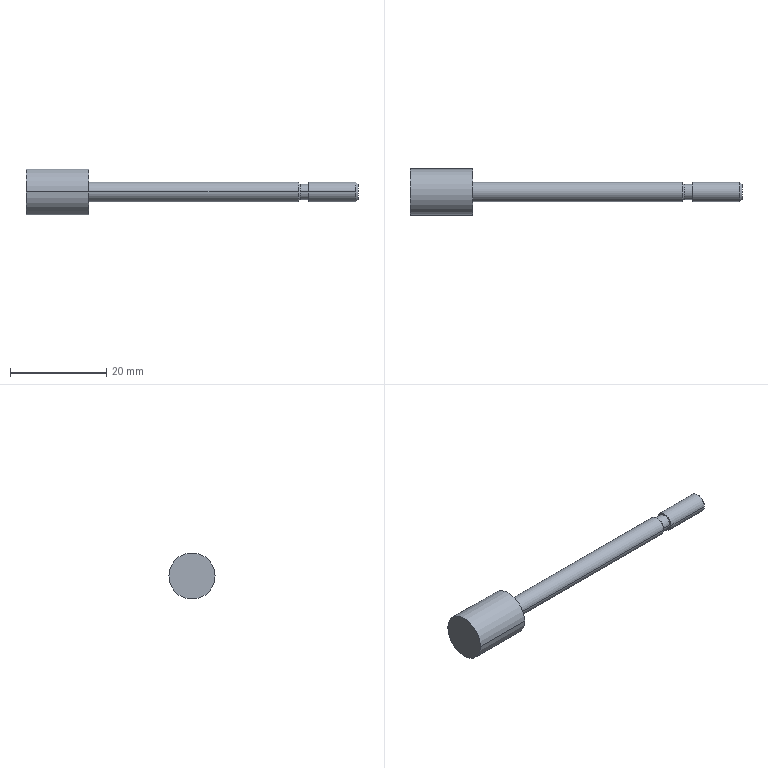Component | SolidWorks | MI10x10U(0)+()-1_MI 10x10-U_r-1 | 1 solid | 16 faces | box 69 x 9.6 x 9.6 mm | volume 1635 mm3 | cylinder 8 | cone 4 | plane 4 | commonest cylinder face diameters 4 x4 9.6 x2 3.2 x2
build123d program:
from build123d import *


with BuildPart() as part:
    # Sketch1 → Revolve1 (revolve)
    with BuildSketch(Plane.XY, mode=Mode.PRIVATE) as revolve1_sk:
        Polygon((-28, 0), (-28, 1.571), (-27.57, 2), (-17.8, 2), (-17.8, 1.6), (-16, 1.6), (-15.6, 2), (28, 2), (28, 4.8), (41, 4.8), (41, 0), align=None)
    revolve(revolve1_sk.sketch.rotate(Axis((41, 0, 0), (-1, 0, 0)), 270), axis=Axis((41, 0, 0), (-1, 0, 0)))


solid = part.part

# Placed as in the assembly
solid = solid.moved(Location((-19.294, 30.452, 72.77), (-180, 0, 180)))
STEP:
#1=COLOUR_RGB('',0.7922,0.8196,0.9333);
#2=FILL_AREA_STYLE_COLOUR('',#1);
#3=FILL_AREA_STYLE('',(#2));
#4=SURFACE_STYLE_FILL_AREA(#3);
#5=SURFACE_SIDE_STYLE('',(#4));
#6=SURFACE_STYLE_USAGE(.BOTH.,#5);
#7=PRESENTATION_STYLE_ASSIGNMENT((#6));
#8=CARTESIAN_POINT('',(-2.374,1.388,2.865));
#9=VERTEX_POINT('',#8);
#10=CARTESIAN_POINT('',(-2.374,1.01,2.865));
#11=VERTEX_POINT('',#10);
#12=CARTESIAN_POINT('',(-2.374,1.199,2.865));
#13=DIRECTION('',(1.,-0.,-0.));
#14=DIRECTION('',(0.,1.,0.));
#15=AXIS2_PLACEMENT_3D('',#12,#13,#14);
#16=CIRCLE('',#15,0.189);
#17=EDGE_CURVE('',#9,#11,#16,.T.);
#18=ORIENTED_EDGE('',*,*,#17,.T.);
#19=CARTESIAN_POINT('',(-1.862,1.01,2.865));
#20=VERTEX_POINT('',#19);
#21=CARTESIAN_POINT('',(-2.374,1.01,2.865));
#22=DIRECTION('',(1.,-0.,-0.));
#23=VECTOR('',#22,39.37);
#24=LINE('',#21,#23);
#25=EDGE_CURVE('',#11,#20,#24,.T.);
#26=ORIENTED_EDGE('',*,*,#25,.T.);
#27=CARTESIAN_POINT('',(-1.862,1.388,2.865));
#28=VERTEX_POINT('',#27);
#29=CARTESIAN_POINT('',(-1.862,1.199,2.865));
#30=DIRECTION('',(1.,-0.,-0.));
#31=DIRECTION('',(0.,1.,0.));
#32=AXIS2_PLACEMENT_3D('',#29,#30,#31);
#33=CIRCLE('',#32,0.189);
#34=EDGE_CURVE('',#28,#20,#33,.T.);
#35=ORIENTED_EDGE('',*,*,#34,.F.);
#36=CARTESIAN_POINT('',(-2.374,1.388,2.865));
#37=DIRECTION('',(1.,-0.,-0.));
#38=VECTOR('',#37,39.37);
#39=LINE('',#36,#38);
#40=EDGE_CURVE('',#9,#28,#39,.T.);
#41=ORIENTED_EDGE('',*,*,#40,.F.);
#42=EDGE_LOOP('',(#18,#26,#35,#41));
#43=FACE_OUTER_BOUND('',#42,.T.);
#44=CARTESIAN_POINT('',(-2.374,1.199,2.865));
#45=DIRECTION('',(1.,-0.,-0.));
#46=DIRECTION('',(0.,1.,0.));
#47=AXIS2_PLACEMENT_3D('',#44,#45,#46);
#48=CYLINDRICAL_SURFACE('',#47,0.189);
#49=ADVANCED_FACE('',(#43),#48,.T.);
#50=CARTESIAN_POINT('',(-1.862,1.278,2.865));
#51=VERTEX_POINT('',#50);
#52=CARTESIAN_POINT('',(-1.862,1.12,2.865));
#53=VERTEX_POINT('',#52);
#54=CARTESIAN_POINT('',(-1.862,1.199,2.865));
#55=DIRECTION('',(1.,-0.,-0.));
#56=DIRECTION('',(0.,1.,0.));
#57=AXIS2_PLACEMENT_3D('',#54,#55,#56);
#58=CIRCLE('',#57,0.07874);
#59=EDGE_CURVE('',#51,#53,#58,.T.);
#60=ORIENTED_EDGE('',*,*,#59,.T.);
#61=CARTESIAN_POINT('',(-0.1454,1.12,2.865));
#62=VERTEX_POINT('',#61);
#63=CARTESIAN_POINT('',(-2.374,1.12,2.865));
#64=DIRECTION('',(1.,-0.,-0.));
#65=VECTOR('',#64,39.37);
#66=LINE('',#63,#65);
#67=EDGE_CURVE('',#53,#62,#66,.T.);
#68=ORIENTED_EDGE('',*,*,#67,.T.);
#69=CARTESIAN_POINT('',(-0.1454,1.278,2.865));
#70=VERTEX_POINT('',#69);
#71=CARTESIAN_POINT('',(-0.1454,1.199,2.865));
#72=DIRECTION('',(1.,-0.,-0.));
#73=DIRECTION('',(0.,1.,0.));
#74=AXIS2_PLACEMENT_3D('',#71,#72,#73);
#75=CIRCLE('',#74,0.07874);
#76=EDGE_CURVE('',#70,#62,#75,.T.);
#77=ORIENTED_EDGE('',*,*,#76,.F.);
#78=CARTESIAN_POINT('',(-2.374,1.278,2.865));
#79=DIRECTION('',(1.,-0.,-0.));
#80=VECTOR('',#79,39.37);
#81=LINE('',#78,#80);
#82=EDGE_CURVE('',#51,#70,#81,.T.);
#83=ORIENTED_EDGE('',*,*,#82,.F.);
#84=EDGE_LOOP('',(#60,#68,#77,#83));
#85=FACE_OUTER_BOUND('',#84,.T.);
#86=CARTESIAN_POINT('',(-2.374,1.199,2.865));
#87=DIRECTION('',(1.,-0.,-0.));
#88=DIRECTION('',(0.,1.,0.));
#89=AXIS2_PLACEMENT_3D('',#86,#87,#88);
#90=CYLINDRICAL_SURFACE('',#89,0.07874);
#91=ADVANCED_FACE('',(#85),#90,.T.);
#92=CARTESIAN_POINT('',(-0.1297,1.262,2.865));
#93=VERTEX_POINT('',#92);
#94=CARTESIAN_POINT('',(-0.1297,1.136,2.865));
#95=VERTEX_POINT('',#94);
#96=CARTESIAN_POINT('',(-0.1297,1.199,2.865));
#97=DIRECTION('',(1.,-0.,-0.));
#98=DIRECTION('',(0.,1.,0.));
#99=AXIS2_PLACEMENT_3D('',#96,#97,#98);
#100=CIRCLE('',#99,0.06299);
#101=EDGE_CURVE('',#93,#95,#100,.T.);
#102=ORIENTED_EDGE('',*,*,#101,.F.);
#103=CARTESIAN_POINT('',(-0.1454,1.278,2.865));
#104=DIRECTION('',(-0.7071,0.7071,0.));
#105=VECTOR('',#104,39.37);
#106=LINE('',#103,#105);
#107=EDGE_CURVE('',#93,#70,#106,.T.);
#108=ORIENTED_EDGE('',*,*,#107,.T.);
#109=ORIENTED_EDGE('',*,*,#76,.T.);
#110=CARTESIAN_POINT('',(-0.1454,1.12,2.865));
#111=DIRECTION('',(-0.7071,-0.7071,-0.));
#112=VECTOR('',#111,39.37);
#113=LINE('',#110,#112);
#114=EDGE_CURVE('',#95,#62,#113,.T.);
#115=ORIENTED_EDGE('',*,*,#114,.F.);
#116=EDGE_LOOP('',(#102,#108,#109,#115));
#117=FACE_OUTER_BOUND('',#116,.T.);
#118=CARTESIAN_POINT('',(-0.1454,1.199,2.865));
#119=DIRECTION('',(-1.,0.,0.));
#120=DIRECTION('',(-0.,-1.,0.));
#121=AXIS2_PLACEMENT_3D('',#118,#119,#120);
#122=CONICAL_SURFACE('',#121,0.07874,0.7854);
#123=ADVANCED_FACE('',(#117),#122,.T.);
#124=ORIENTED_EDGE('',*,*,#101,.T.);
#125=CARTESIAN_POINT('',(-0.05882,1.136,2.865));
#126=VERTEX_POINT('',#125);
#127=CARTESIAN_POINT('',(-2.374,1.136,2.865));
#128=DIRECTION('',(1.,-0.,-0.));
#129=VECTOR('',#128,39.37);
#130=LINE('',#127,#129);
#131=EDGE_CURVE('',#95,#126,#130,.T.);
#132=ORIENTED_EDGE('',*,*,#131,.T.);
#133=CARTESIAN_POINT('',(-0.05882,1.262,2.865));
#134=VERTEX_POINT('',#133);
#135=CARTESIAN_POINT('',(-0.05882,1.199,2.865));
#136=DIRECTION('',(1.,-0.,-0.));
#137=DIRECTION('',(0.,1.,0.));
#138=AXIS2_PLACEMENT_3D('',#135,#136,#137);
#139=CIRCLE('',#138,0.06299);
#140=EDGE_CURVE('',#134,#126,#139,.T.);
#141=ORIENTED_EDGE('',*,*,#140,.F.);
#142=CARTESIAN_POINT('',(-2.374,1.262,2.865));
#143=DIRECTION('',(1.,-0.,-0.));
#144=VECTOR('',#143,39.37);
#145=LINE('',#142,#144);
#146=EDGE_CURVE('',#93,#134,#145,.T.);
#147=ORIENTED_EDGE('',*,*,#146,.F.);
#148=EDGE_LOOP('',(#124,#132,#141,#147));
#149=FACE_OUTER_BOUND('',#148,.T.);
#150=CARTESIAN_POINT('',(-2.374,1.199,2.865));
#151=DIRECTION('',(1.,-0.,-0.));
#152=DIRECTION('',(0.,1.,0.));
#153=AXIS2_PLACEMENT_3D('',#150,#151,#152);
#154=CYLINDRICAL_SURFACE('',#153,0.06299);
#155=ADVANCED_FACE('',(#149),#154,.T.);
#156=CARTESIAN_POINT('',(-0.05882,1.278,2.865));
#157=VERTEX_POINT('',#156);
#158=CARTESIAN_POINT('',(-0.05882,1.12,2.865));
#159=VERTEX_POINT('',#158);
#160=CARTESIAN_POINT('',(-0.05882,1.199,2.865));
#161=DIRECTION('',(1.,-0.,-0.));
#162=DIRECTION('',(0.,1.,0.));
#163=AXIS2_PLACEMENT_3D('',#160,#161,#162);
#164=CIRCLE('',#163,0.07874);
#165=EDGE_CURVE('',#157,#159,#164,.T.);
#166=ORIENTED_EDGE('',*,*,#165,.T.);
#167=CARTESIAN_POINT('',(0.3258,1.12,2.865));
#168=VERTEX_POINT('',#167);
#169=CARTESIAN_POINT('',(-2.374,1.12,2.865));
#170=DIRECTION('',(1.,-0.,-0.));
#171=VECTOR('',#170,39.37);
#172=LINE('',#169,#171);
#173=EDGE_CURVE('',#159,#168,#172,.T.);
#174=ORIENTED_EDGE('',*,*,#173,.T.);
#175=CARTESIAN_POINT('',(0.3258,1.278,2.865));
#176=VERTEX_POINT('',#175);
#177=CARTESIAN_POINT('',(0.3258,1.199,2.865));
#178=DIRECTION('',(1.,-0.,-0.));
#179=DIRECTION('',(0.,1.,0.));
#180=AXIS2_PLACEMENT_3D('',#177,#178,#179);
#181=CIRCLE('',#180,0.07874);
#182=EDGE_CURVE('',#176,#168,#181,.T.);
#183=ORIENTED_EDGE('',*,*,#182,.F.);
#184=CARTESIAN_POINT('',(-2.374,1.278,2.865));
#185=DIRECTION('',(1.,-0.,-0.));
#186=VECTOR('',#185,39.37);
#187=LINE('',#184,#186);
#188=EDGE_CURVE('',#157,#176,#187,.T.);
#189=ORIENTED_EDGE('',*,*,#188,.F.);
#190=EDGE_LOOP('',(#166,#174,#183,#189));
#191=FACE_OUTER_BOUND('',#190,.T.);
#192=CARTESIAN_POINT('',(-2.374,1.199,2.865));
#193=DIRECTION('',(1.,-0.,-0.));
#194=DIRECTION('',(0.,1.,0.));
#195=AXIS2_PLACEMENT_3D('',#192,#193,#194);
#196=CYLINDRICAL_SURFACE('',#195,0.07874);
#197=ADVANCED_FACE('',(#191),#196,.T.);
#198=CARTESIAN_POINT('',(0.3428,1.261,2.865));
#199=VERTEX_POINT('',#198);
#200=CARTESIAN_POINT('',(0.3428,1.137,2.865));
#201=VERTEX_POINT('',#200);
#202=CARTESIAN_POINT('',(0.3428,1.199,2.865));
#203=DIRECTION('',(1.,-0.,-0.));
#204=DIRECTION('',(0.,1.,0.));
#205=AXIS2_PLACEMENT_3D('',#202,#203,#204);
#206=CIRCLE('',#205,0.06183);
#207=EDGE_CURVE('',#199,#201,#206,.T.);
#208=ORIENTED_EDGE('',*,*,#207,.F.);
#209=CARTESIAN_POINT('',(0.3258,1.278,2.865));
#210=DIRECTION('',(-0.7071,0.7071,0.));
#211=VECTOR('',#210,39.37);
#212=LINE('',#209,#211);
#213=EDGE_CURVE('',#199,#176,#212,.T.);
#214=ORIENTED_EDGE('',*,*,#213,.T.);
#215=ORIENTED_EDGE('',*,*,#182,.T.);
#216=CARTESIAN_POINT('',(0.3258,1.12,2.865));
#217=DIRECTION('',(-0.7071,-0.7071,-0.));
#218=VECTOR('',#217,39.37);
#219=LINE('',#216,#218);
#220=EDGE_CURVE('',#201,#168,#219,.T.);
#221=ORIENTED_EDGE('',*,*,#220,.F.);
#222=EDGE_LOOP('',(#208,#214,#215,#221));
#223=FACE_OUTER_BOUND('',#222,.T.);
#224=CARTESIAN_POINT('',(0.3258,1.199,2.865));
#225=DIRECTION('',(-1.,0.,0.));
#226=DIRECTION('',(0.,-1.,0.));
#227=AXIS2_PLACEMENT_3D('',#224,#225,#226);
#228=CONICAL_SURFACE('',#227,0.07874,0.7854);
#229=ADVANCED_FACE('',(#223),#228,.T.);
#230=CARTESIAN_POINT('',(0.3428,1.199,2.865));
#231=DIRECTION('',(1.,-0.,-0.));
#232=DIRECTION('',(0.,1.,0.));
#233=AXIS2_PLACEMENT_3D('',#230,#231,#232);
#234=CIRCLE('',#233,0.06183);
#235=EDGE_CURVE('',#201,#199,#234,.T.);
#236=ORIENTED_EDGE('',*,*,#235,.T.);
#237=ORIENTED_EDGE('',*,*,#207,.T.);
#238=EDGE_LOOP('',(#236,#237));
#239=FACE_OUTER_BOUND('',#238,.T.);
#240=CARTESIAN_POINT('',(0.3428,1.199,2.865));
#241=DIRECTION('',(-1.,0.,0.));
#242=DIRECTION('',(-0.,-1.,-0.));
#243=AXIS2_PLACEMENT_3D('',#240,#241,#242);
#244=PLANE('',#243);
#245=ADVANCED_FACE('',(#239),#244,.F.);
#246=ORIENTED_EDGE('',*,*,#213,.F.);
#247=ORIENTED_EDGE('',*,*,#235,.F.);
#248=ORIENTED_EDGE('',*,*,#220,.T.);
#249=CARTESIAN_POINT('',(0.3258,1.199,2.865));
#250=DIRECTION('',(1.,-0.,-0.));
#251=DIRECTION('',(0.,1.,0.));
#252=AXIS2_PLACEMENT_3D('',#249,#250,#251);
#253=CIRCLE('',#252,0.07874);
#254=EDGE_CURVE('',#168,#176,#253,.T.);
#255=ORIENTED_EDGE('',*,*,#254,.T.);
#256=EDGE_LOOP('',(#246,#247,#248,#255));
#257=FACE_OUTER_BOUND('',#256,.T.);
#258=CARTESIAN_POINT('',(0.3258,1.199,2.865));
#259=DIRECTION('',(-1.,0.,0.));
#260=DIRECTION('',(0.,-1.,0.));
#261=AXIS2_PLACEMENT_3D('',#258,#259,#260);
#262=CONICAL_SURFACE('',#261,0.07874,0.7854);
#263=ADVANCED_FACE('',(#257),#262,.T.);
#264=ORIENTED_EDGE('',*,*,#173,.F.);
#265=CARTESIAN_POINT('',(-0.05882,1.199,2.865));
#266=DIRECTION('',(1.,-0.,-0.));
#267=DIRECTION('',(0.,1.,0.));
#268=AXIS2_PLACEMENT_3D('',#265,#266,#267);
#269=CIRCLE('',#268,0.07874);
#270=EDGE_CURVE('',#159,#157,#269,.T.);
#271=ORIENTED_EDGE('',*,*,#270,.T.);
#272=ORIENTED_EDGE('',*,*,#188,.T.);
#273=ORIENTED_EDGE('',*,*,#254,.F.);
#274=EDGE_LOOP('',(#264,#271,#272,#273));
#275=FACE_OUTER_BOUND('',#274,.T.);
#276=CARTESIAN_POINT('',(-2.374,1.199,2.865));
#277=DIRECTION('',(1.,-0.,-0.));
#278=DIRECTION('',(0.,1.,0.));
#279=AXIS2_PLACEMENT_3D('',#276,#277,#278);
#280=CYLINDRICAL_SURFACE('',#279,0.07874);
#281=ADVANCED_FACE('',(#275),#280,.T.);
#282=ORIENTED_EDGE('',*,*,#165,.F.);
#283=ORIENTED_EDGE('',*,*,#270,.F.);
#284=EDGE_LOOP('',(#282,#283));
#285=FACE_OUTER_BOUND('',#284,.T.);
#286=ORIENTED_EDGE('',*,*,#140,.T.);
#287=CARTESIAN_POINT('',(-0.05882,1.199,2.865));
#288=DIRECTION('',(1.,-0.,-0.));
#289=DIRECTION('',(0.,1.,0.));
#290=AXIS2_PLACEMENT_3D('',#287,#288,#289);
#291=CIRCLE('',#290,0.06299);
#292=EDGE_CURVE('',#126,#134,#291,.T.);
#293=ORIENTED_EDGE('',*,*,#292,.T.);
#294=EDGE_LOOP('',(#286,#293));
#295=FACE_BOUND('',#294,.T.);
#296=CARTESIAN_POINT('',(-0.05882,1.199,2.944));
#297=DIRECTION('',(1.,-0.,-0.));
#298=DIRECTION('',(0.,1.,0.));
#299=AXIS2_PLACEMENT_3D('',#296,#297,#298);
#300=PLANE('',#299);
#301=ADVANCED_FACE('',(#285,#295),#300,.F.);
#302=ORIENTED_EDGE('',*,*,#131,.F.);
#303=CARTESIAN_POINT('',(-0.1297,1.199,2.865));
#304=DIRECTION('',(1.,-0.,-0.));
#305=DIRECTION('',(0.,1.,0.));
#306=AXIS2_PLACEMENT_3D('',#303,#304,#305);
#307=CIRCLE('',#306,0.06299);
#308=EDGE_CURVE('',#95,#93,#307,.T.);
#309=ORIENTED_EDGE('',*,*,#308,.T.);
#310=ORIENTED_EDGE('',*,*,#146,.T.);
#311=ORIENTED_EDGE('',*,*,#292,.F.);
#312=EDGE_LOOP('',(#302,#309,#310,#311));
#313=FACE_OUTER_BOUND('',#312,.T.);
#314=CARTESIAN_POINT('',(-2.374,1.199,2.865));
#315=DIRECTION('',(1.,-0.,-0.));
#316=DIRECTION('',(0.,1.,0.));
#317=AXIS2_PLACEMENT_3D('',#314,#315,#316);
#318=CYLINDRICAL_SURFACE('',#317,0.06299);
#319=ADVANCED_FACE('',(#313),#318,.T.);
#320=ORIENTED_EDGE('',*,*,#107,.F.);
#321=ORIENTED_EDGE('',*,*,#308,.F.);
#322=ORIENTED_EDGE('',*,*,#114,.T.);
#323=CARTESIAN_POINT('',(-0.1454,1.199,2.865));
#324=DIRECTION('',(1.,-0.,-0.));
#325=DIRECTION('',(0.,1.,0.));
#326=AXIS2_PLACEMENT_3D('',#323,#324,#325);
#327=CIRCLE('',#326,0.07874);
#328=EDGE_CURVE('',#62,#70,#327,.T.);
#329=ORIENTED_EDGE('',*,*,#328,.T.);
#330=EDGE_LOOP('',(#320,#321,#322,#329));
#331=FACE_OUTER_BOUND('',#330,.T.);
#332=CARTESIAN_POINT('',(-0.1454,1.199,2.865));
#333=DIRECTION('',(-1.,0.,0.));
#334=DIRECTION('',(-0.,-1.,0.));
#335=AXIS2_PLACEMENT_3D('',#332,#333,#334);
#336=CONICAL_SURFACE('',#335,0.07874,0.7854);
#337=ADVANCED_FACE('',(#331),#336,.T.);
#338=ORIENTED_EDGE('',*,*,#67,.F.);
#339=CARTESIAN_POINT('',(-1.862,1.199,2.865));
#340=DIRECTION('',(1.,-0.,-0.));
#341=DIRECTION('',(0.,1.,0.));
#342=AXIS2_PLACEMENT_3D('',#339,#340,#341);
#343=CIRCLE('',#342,0.07874);
#344=EDGE_CURVE('',#53,#51,#343,.T.);
#345=ORIENTED_EDGE('',*,*,#344,.T.);
#346=ORIENTED_EDGE('',*,*,#82,.T.);
#347=ORIENTED_EDGE('',*,*,#328,.F.);
#348=EDGE_LOOP('',(#338,#345,#346,#347));
#349=FACE_OUTER_BOUND('',#348,.T.);
#350=CARTESIAN_POINT('',(-2.374,1.199,2.865));
#351=DIRECTION('',(1.,-0.,-0.));
#352=DIRECTION('',(0.,1.,0.));
#353=AXIS2_PLACEMENT_3D('',#350,#351,#352);
#354=CYLINDRICAL_SURFACE('',#353,0.07874);
#355=ADVANCED_FACE('',(#349),#354,.T.);
#356=ORIENTED_EDGE('',*,*,#59,.F.);
#357=ORIENTED_EDGE('',*,*,#344,.F.);
#358=EDGE_LOOP('',(#356,#357));
#359=FACE_BOUND('',#358,.T.);
#360=ORIENTED_EDGE('',*,*,#34,.T.);
#361=CARTESIAN_POINT('',(-1.862,1.199,2.865));
#362=DIRECTION('',(1.,-0.,-0.));
#363=DIRECTION('',(0.,1.,0.));
#364=AXIS2_PLACEMENT_3D('',#361,#362,#363);
#365=CIRCLE('',#364,0.189);
#366=EDGE_CURVE('',#20,#28,#365,.T.);
#367=ORIENTED_EDGE('',*,*,#366,.T.);
#368=EDGE_LOOP('',(#360,#367));
#369=FACE_OUTER_BOUND('',#368,.T.);
#370=CARTESIAN_POINT('',(-1.862,1.199,2.944));
#371=DIRECTION('',(-1.,0.,0.));
#372=DIRECTION('',(-0.,-1.,-0.));
#373=AXIS2_PLACEMENT_3D('',#370,#371,#372);
#374=PLANE('',#373);
#375=ADVANCED_FACE('',(#359,#369),#374,.F.);
#376=ORIENTED_EDGE('',*,*,#25,.F.);
#377=CARTESIAN_POINT('',(-2.374,1.199,2.865));
#378=DIRECTION('',(1.,-0.,-0.));
#379=DIRECTION('',(0.,1.,0.));
#380=AXIS2_PLACEMENT_3D('',#377,#378,#379);
#381=CIRCLE('',#380,0.189);
#382=EDGE_CURVE('',#11,#9,#381,.T.);
#383=ORIENTED_EDGE('',*,*,#382,.T.);
#384=ORIENTED_EDGE('',*,*,#40,.T.);
#385=ORIENTED_EDGE('',*,*,#366,.F.);
#386=EDGE_LOOP('',(#376,#383,#384,#385));
#387=FACE_OUTER_BOUND('',#386,.T.);
#388=CARTESIAN_POINT('',(-2.374,1.199,2.865));
#389=DIRECTION('',(1.,-0.,-0.));
#390=DIRECTION('',(0.,1.,0.));
#391=AXIS2_PLACEMENT_3D('',#388,#389,#390);
#392=CYLINDRICAL_SURFACE('',#391,0.189);
#393=ADVANCED_FACE('',(#387),#392,.T.);
#394=ORIENTED_EDGE('',*,*,#17,.F.);
#395=ORIENTED_EDGE('',*,*,#382,.F.);
#396=EDGE_LOOP('',(#394,#395));
#397=FACE_OUTER_BOUND('',#396,.T.);
#398=CARTESIAN_POINT('',(-2.374,1.199,3.054));
#399=DIRECTION('',(1.,-0.,-0.));
#400=DIRECTION('',(0.,1.,0.));
#401=AXIS2_PLACEMENT_3D('',#398,#399,#400);
#402=PLANE('',#401);
#403=ADVANCED_FACE('',(#397),#402,.F.);
#404=CLOSED_SHELL('',(#49,#91,#123,#155,#197,#229,#245,#263,#281,#301,#319,#337,#355,#375,#393,#403));
#405=MANIFOLD_SOLID_BREP('',#404);
#406=STYLED_ITEM('',(#7),#405);
#407=(LENGTH_UNIT()NAMED_UNIT(*)SI_UNIT($,.METRE.));
#408=LENGTH_MEASURE_WITH_UNIT(LENGTH_MEASURE(0.0254),#407);
#409=DIMENSIONAL_EXPONENTS(1.,0.,0.,0.,0.,0.,0.);
#410=(CONVERSION_BASED_UNIT('',#408)LENGTH_UNIT()NAMED_UNIT(#409));
#411=UNCERTAINTY_MEASURE_WITH_UNIT(LENGTH_MEASURE(0.00001),#410,'','');
#412=(NAMED_UNIT(*)PLANE_ANGLE_UNIT()SI_UNIT($,.RADIAN.));
#413=(NAMED_UNIT(*)SI_UNIT($,.STERADIAN.)SOLID_ANGLE_UNIT());
#414=(GEOMETRIC_REPRESENTATION_CONTEXT(3)GLOBAL_UNCERTAINTY_ASSIGNED_CONTEXT((#411))GLOBAL_UNIT_ASSIGNED_CONTEXT((#410,#412,#413))REPRESENTATION_CONTEXT('',''));
#415=MECHANICAL_DESIGN_GEOMETRIC_PRESENTATION_REPRESENTATION('',(#406),#414);
#416=CARTESIAN_POINT('',(0.,0.,0.));
#417=DIRECTION('',(0.,0.,1.));
#418=DIRECTION('',(1.,0.,0.));
#419=AXIS2_PLACEMENT_3D('',#416,#417,#418);
#420=(LENGTH_UNIT()NAMED_UNIT(*)SI_UNIT($,.METRE.));
#421=LENGTH_MEASURE_WITH_UNIT(LENGTH_MEASURE(0.0254),#420);
#422=DIMENSIONAL_EXPONENTS(1.,0.,0.,0.,0.,0.,0.);
#423=(CONVERSION_BASED_UNIT('',#421)LENGTH_UNIT()NAMED_UNIT(#422));
#424=UNCERTAINTY_MEASURE_WITH_UNIT(LENGTH_MEASURE(0.00001),#423,'','');
#425=(NAMED_UNIT(*)PLANE_ANGLE_UNIT()SI_UNIT($,.RADIAN.));
#426=(NAMED_UNIT(*)SI_UNIT($,.STERADIAN.)SOLID_ANGLE_UNIT());
#427=(GEOMETRIC_REPRESENTATION_CONTEXT(3)GLOBAL_UNCERTAINTY_ASSIGNED_CONTEXT((#424))GLOBAL_UNIT_ASSIGNED_CONTEXT((#423,#425,#426))REPRESENTATION_CONTEXT('',''));
#428=ADVANCED_BREP_SHAPE_REPRESENTATION('',(#405,#419),#427);
#429=PRESENTATION_LAYER_ASSIGNMENT('','',(#406));